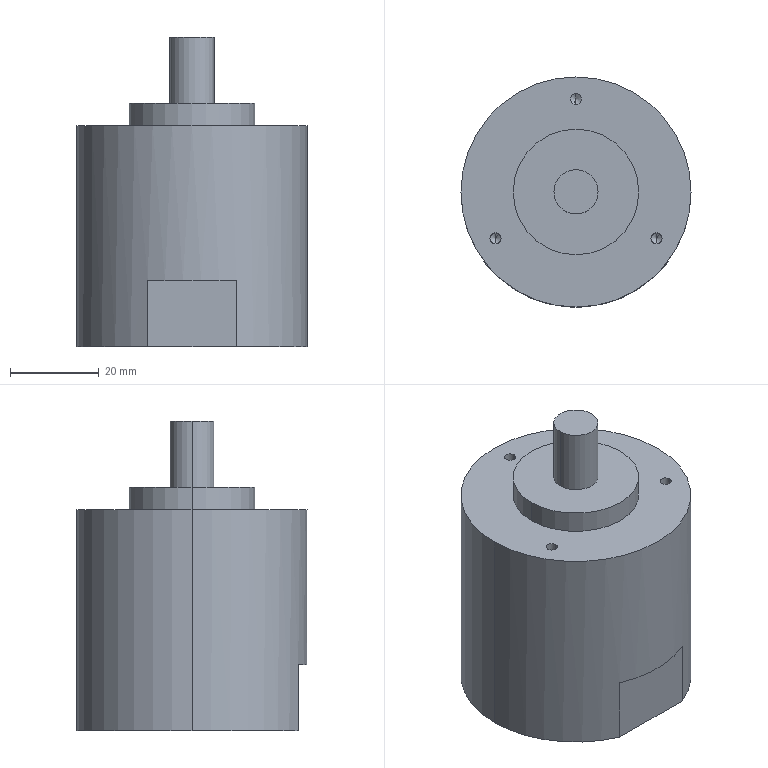Component | SolidWorks | YC1-250-09SecondDropAssembly-1_Sensor-1 | 1 solid | 24 faces | box 52 x 52 x 70 mm | volume 109999 mm3 | cylinder 12 | cone 6 | plane 6 | commonest cylinder face diameters 2.5 x6 52 x2 28.4 x2 10 x2 | material Plain Carbon Steel
STEP:
#1=COLOUR_RGB('',0.7922,0.8196,0.9333);
#2=FILL_AREA_STYLE_COLOUR('',#1);
#3=FILL_AREA_STYLE('',(#2));
#4=SURFACE_STYLE_FILL_AREA(#3);
#5=SURFACE_SIDE_STYLE('',(#4));
#6=SURFACE_STYLE_USAGE(.BOTH.,#5);
#7=PRESENTATION_STYLE_ASSIGNMENT((#6));
#8=CARTESIAN_POINT('',(1.024,131.693,-45.748));
#9=VERTEX_POINT('',#8);
#10=CARTESIAN_POINT('',(-1.024,131.693,-45.748));
#11=VERTEX_POINT('',#10);
#12=CARTESIAN_POINT('',(0.,131.693,-45.748));
#13=DIRECTION('',(0.,-0.,1.));
#14=DIRECTION('',(1.,0.,0.));
#15=AXIS2_PLACEMENT_3D('',#12,#13,#14);
#16=CIRCLE('',#15,1.024);
#17=EDGE_CURVE('',#9,#11,#16,.T.);
#18=ORIENTED_EDGE('',*,*,#17,.T.);
#19=CARTESIAN_POINT('',(-1.024,131.693,-43.78));
#20=VERTEX_POINT('',#19);
#21=CARTESIAN_POINT('',(-1.024,131.693,-39.81));
#22=DIRECTION('',(0.,-0.,1.));
#23=VECTOR('',#22,39.37);
#24=LINE('',#21,#23);
#25=EDGE_CURVE('',#11,#20,#24,.T.);
#26=ORIENTED_EDGE('',*,*,#25,.T.);
#27=CARTESIAN_POINT('',(1.024,131.693,-43.78));
#28=VERTEX_POINT('',#27);
#29=CARTESIAN_POINT('',(0.,131.693,-43.78));
#30=DIRECTION('',(-0.,0.,-1.));
#31=DIRECTION('',(1.,0.,0.));
#32=AXIS2_PLACEMENT_3D('',#29,#30,#31);
#33=CIRCLE('',#32,1.024);
#34=EDGE_CURVE('',#20,#28,#33,.T.);
#35=ORIENTED_EDGE('',*,*,#34,.T.);
#36=CARTESIAN_POINT('',(1.024,131.693,-39.81));
#37=DIRECTION('',(0.,-0.,1.));
#38=VECTOR('',#37,39.37);
#39=LINE('',#36,#38);
#40=EDGE_CURVE('',#9,#28,#39,.T.);
#41=ORIENTED_EDGE('',*,*,#40,.F.);
#42=EDGE_LOOP('',(#18,#26,#35,#41));
#43=FACE_OUTER_BOUND('',#42,.T.);
#44=CARTESIAN_POINT('',(0.,131.693,-39.81));
#45=DIRECTION('',(0.,-0.,1.));
#46=DIRECTION('',(1.,0.,0.));
#47=AXIS2_PLACEMENT_3D('',#44,#45,#46);
#48=CYLINDRICAL_SURFACE('',#47,1.024);
#49=ADVANCED_FACE('',(#43),#48,.T.);
#50=CARTESIAN_POINT('',(-0.5591,131.693,-43.78));
#51=VERTEX_POINT('',#50);
#52=CARTESIAN_POINT('',(0.5591,131.693,-43.78));
#53=VERTEX_POINT('',#52);
#54=CARTESIAN_POINT('',(0.,131.693,-43.78));
#55=DIRECTION('',(-0.,0.,-1.));
#56=DIRECTION('',(1.,0.,0.));
#57=AXIS2_PLACEMENT_3D('',#54,#55,#56);
#58=CIRCLE('',#57,0.5591);
#59=EDGE_CURVE('',#51,#53,#58,.T.);
#60=ORIENTED_EDGE('',*,*,#59,.F.);
#61=CARTESIAN_POINT('',(-0.5591,131.693,-43.583));
#62=VERTEX_POINT('',#61);
#63=CARTESIAN_POINT('',(-0.5591,131.693,-39.81));
#64=DIRECTION('',(0.,-0.,1.));
#65=VECTOR('',#64,39.37);
#66=LINE('',#63,#65);
#67=EDGE_CURVE('',#51,#62,#66,.T.);
#68=ORIENTED_EDGE('',*,*,#67,.T.);
#69=CARTESIAN_POINT('',(0.5591,131.693,-43.583));
#70=VERTEX_POINT('',#69);
#71=CARTESIAN_POINT('',(0.,131.693,-43.583));
#72=DIRECTION('',(-0.,0.,-1.));
#73=DIRECTION('',(1.,0.,0.));
#74=AXIS2_PLACEMENT_3D('',#71,#72,#73);
#75=CIRCLE('',#74,0.5591);
#76=EDGE_CURVE('',#62,#70,#75,.T.);
#77=ORIENTED_EDGE('',*,*,#76,.T.);
#78=CARTESIAN_POINT('',(0.5591,131.693,-39.81));
#79=DIRECTION('',(0.,-0.,1.));
#80=VECTOR('',#79,39.37);
#81=LINE('',#78,#80);
#82=EDGE_CURVE('',#53,#70,#81,.T.);
#83=ORIENTED_EDGE('',*,*,#82,.F.);
#84=EDGE_LOOP('',(#60,#68,#77,#83));
#85=FACE_OUTER_BOUND('',#84,.T.);
#86=CARTESIAN_POINT('',(0.,131.693,-39.81));
#87=DIRECTION('',(0.,-0.,1.));
#88=DIRECTION('',(1.,0.,0.));
#89=AXIS2_PLACEMENT_3D('',#86,#87,#88);
#90=CYLINDRICAL_SURFACE('',#89,0.5591);
#91=ADVANCED_FACE('',(#85),#90,.T.);
#92=CARTESIAN_POINT('',(0.6668,131.28,-44.114));
#93=VERTEX_POINT('',#92);
#94=CARTESIAN_POINT('',(0.716,131.23,-44.114));
#95=VERTEX_POINT('',#94);
#96=CARTESIAN_POINT('',(0.716,131.28,-44.114));
#97=DIRECTION('',(0.,-0.,1.));
#98=DIRECTION('',(1.,0.,0.));
#99=AXIS2_PLACEMENT_3D('',#96,#97,#98);
#100=CIRCLE('',#99,0.04921);
#101=EDGE_CURVE('',#93,#95,#100,.T.);
#102=ORIENTED_EDGE('',*,*,#101,.F.);
#103=CARTESIAN_POINT('',(0.6668,131.28,-43.78));
#104=VERTEX_POINT('',#103);
#105=CARTESIAN_POINT('',(0.6668,131.28,-43.78));
#106=DIRECTION('',(0.,-0.,1.));
#107=VECTOR('',#106,39.37);
#108=LINE('',#105,#107);
#109=EDGE_CURVE('',#93,#104,#108,.T.);
#110=ORIENTED_EDGE('',*,*,#109,.T.);
#111=CARTESIAN_POINT('',(0.7652,131.28,-43.78));
#112=VERTEX_POINT('',#111);
#113=CARTESIAN_POINT('',(0.716,131.28,-43.78));
#114=DIRECTION('',(-0.,0.,-1.));
#115=DIRECTION('',(1.,0.,0.));
#116=AXIS2_PLACEMENT_3D('',#113,#114,#115);
#117=CIRCLE('',#116,0.04921);
#118=EDGE_CURVE('',#112,#104,#117,.T.);
#119=ORIENTED_EDGE('',*,*,#118,.F.);
#120=CARTESIAN_POINT('',(0.7652,131.28,-44.114));
#121=VERTEX_POINT('',#120);
#122=CARTESIAN_POINT('',(0.7652,131.28,-43.78));
#123=DIRECTION('',(0.,-0.,1.));
#124=VECTOR('',#123,39.37);
#125=LINE('',#122,#124);
#126=EDGE_CURVE('',#121,#112,#125,.T.);
#127=ORIENTED_EDGE('',*,*,#126,.F.);
#128=CARTESIAN_POINT('',(0.716,131.28,-44.114));
#129=DIRECTION('',(0.,-0.,1.));
#130=DIRECTION('',(1.,0.,0.));
#131=AXIS2_PLACEMENT_3D('',#128,#129,#130);
#132=CIRCLE('',#131,0.04921);
#133=EDGE_CURVE('',#95,#121,#132,.T.);
#134=ORIENTED_EDGE('',*,*,#133,.F.);
#135=EDGE_LOOP('',(#102,#110,#119,#127,#134));
#136=FACE_OUTER_BOUND('',#135,.T.);
#137=CARTESIAN_POINT('',(0.716,131.28,-43.78));
#138=DIRECTION('',(0.,-0.,1.));
#139=DIRECTION('',(1.,0.,0.));
#140=AXIS2_PLACEMENT_3D('',#137,#138,#139);
#141=CYLINDRICAL_SURFACE('',#140,0.04921);
#142=ADVANCED_FACE('',(#136),#141,.F.);
#143=CARTESIAN_POINT('',(-0.04921,132.52,-44.114));
#144=VERTEX_POINT('',#143);
#145=CARTESIAN_POINT('',(0.,132.47,-44.114));
#146=VERTEX_POINT('',#145);
#147=CARTESIAN_POINT('',(0.,132.52,-44.114));
#148=DIRECTION('',(0.,-0.,1.));
#149=DIRECTION('',(1.,0.,0.));
#150=AXIS2_PLACEMENT_3D('',#147,#148,#149);
#151=CIRCLE('',#150,0.04921);
#152=EDGE_CURVE('',#144,#146,#151,.T.);
#153=ORIENTED_EDGE('',*,*,#152,.F.);
#154=CARTESIAN_POINT('',(-0.04921,132.52,-43.78));
#155=VERTEX_POINT('',#154);
#156=CARTESIAN_POINT('',(-0.04921,132.52,-43.78));
#157=DIRECTION('',(0.,-0.,1.));
#158=VECTOR('',#157,39.37);
#159=LINE('',#156,#158);
#160=EDGE_CURVE('',#144,#155,#159,.T.);
#161=ORIENTED_EDGE('',*,*,#160,.T.);
#162=CARTESIAN_POINT('',(0.04921,132.52,-43.78));
#163=VERTEX_POINT('',#162);
#164=CARTESIAN_POINT('',(0.,132.52,-43.78));
#165=DIRECTION('',(-0.,0.,-1.));
#166=DIRECTION('',(1.,0.,0.));
#167=AXIS2_PLACEMENT_3D('',#164,#165,#166);
#168=CIRCLE('',#167,0.04921);
#169=EDGE_CURVE('',#163,#155,#168,.T.);
#170=ORIENTED_EDGE('',*,*,#169,.F.);
#171=CARTESIAN_POINT('',(0.04921,132.52,-44.114));
#172=VERTEX_POINT('',#171);
#173=CARTESIAN_POINT('',(0.04921,132.52,-43.78));
#174=DIRECTION('',(0.,-0.,1.));
#175=VECTOR('',#174,39.37);
#176=LINE('',#173,#175);
#177=EDGE_CURVE('',#172,#163,#176,.T.);
#178=ORIENTED_EDGE('',*,*,#177,.F.);
#179=CARTESIAN_POINT('',(0.,132.52,-44.114));
#180=DIRECTION('',(0.,-0.,1.));
#181=DIRECTION('',(1.,0.,0.));
#182=AXIS2_PLACEMENT_3D('',#179,#180,#181);
#183=CIRCLE('',#182,0.04921);
#184=EDGE_CURVE('',#146,#172,#183,.T.);
#185=ORIENTED_EDGE('',*,*,#184,.F.);
#186=EDGE_LOOP('',(#153,#161,#170,#178,#185));
#187=FACE_OUTER_BOUND('',#186,.T.);
#188=CARTESIAN_POINT('',(0.,132.52,-43.78));
#189=DIRECTION('',(0.,-0.,1.));
#190=DIRECTION('',(1.,0.,0.));
#191=AXIS2_PLACEMENT_3D('',#188,#189,#190);
#192=CYLINDRICAL_SURFACE('',#191,0.04921);
#193=ADVANCED_FACE('',(#187),#192,.F.);
#194=CARTESIAN_POINT('',(-0.7652,131.28,-44.114));
#195=VERTEX_POINT('',#194);
#196=CARTESIAN_POINT('',(-0.716,131.23,-44.114));
#197=VERTEX_POINT('',#196);
#198=CARTESIAN_POINT('',(-0.716,131.28,-44.114));
#199=DIRECTION('',(0.,-0.,1.));
#200=DIRECTION('',(1.,0.,0.));
#201=AXIS2_PLACEMENT_3D('',#198,#199,#200);
#202=CIRCLE('',#201,0.04921);
#203=EDGE_CURVE('',#195,#197,#202,.T.);
#204=ORIENTED_EDGE('',*,*,#203,.F.);
#205=CARTESIAN_POINT('',(-0.7652,131.28,-43.78));
#206=VERTEX_POINT('',#205);
#207=CARTESIAN_POINT('',(-0.7652,131.28,-43.78));
#208=DIRECTION('',(0.,-0.,1.));
#209=VECTOR('',#208,39.37);
#210=LINE('',#207,#209);
#211=EDGE_CURVE('',#195,#206,#210,.T.);
#212=ORIENTED_EDGE('',*,*,#211,.T.);
#213=CARTESIAN_POINT('',(-0.6668,131.28,-43.78));
#214=VERTEX_POINT('',#213);
#215=CARTESIAN_POINT('',(-0.716,131.28,-43.78));
#216=DIRECTION('',(-0.,0.,-1.));
#217=DIRECTION('',(1.,0.,0.));
#218=AXIS2_PLACEMENT_3D('',#215,#216,#217);
#219=CIRCLE('',#218,0.04921);
#220=EDGE_CURVE('',#214,#206,#219,.T.);
#221=ORIENTED_EDGE('',*,*,#220,.F.);
#222=CARTESIAN_POINT('',(-0.6668,131.28,-44.114));
#223=VERTEX_POINT('',#222);
#224=CARTESIAN_POINT('',(-0.6668,131.28,-43.78));
#225=DIRECTION('',(0.,-0.,1.));
#226=VECTOR('',#225,39.37);
#227=LINE('',#224,#226);
#228=EDGE_CURVE('',#223,#214,#227,.T.);
#229=ORIENTED_EDGE('',*,*,#228,.F.);
#230=CARTESIAN_POINT('',(-0.716,131.28,-44.114));
#231=DIRECTION('',(0.,-0.,1.));
#232=DIRECTION('',(1.,0.,0.));
#233=AXIS2_PLACEMENT_3D('',#230,#231,#232);
#234=CIRCLE('',#233,0.04921);
#235=EDGE_CURVE('',#197,#223,#234,.T.);
#236=ORIENTED_EDGE('',*,*,#235,.F.);
#237=EDGE_LOOP('',(#204,#212,#221,#229,#236));
#238=FACE_OUTER_BOUND('',#237,.T.);
#239=CARTESIAN_POINT('',(-0.716,131.28,-43.78));
#240=DIRECTION('',(0.,-0.,1.));
#241=DIRECTION('',(1.,0.,0.));
#242=AXIS2_PLACEMENT_3D('',#239,#240,#241);
#243=CYLINDRICAL_SURFACE('',#242,0.04921);
#244=ADVANCED_FACE('',(#238),#243,.F.);
#245=CARTESIAN_POINT('',(0.716,131.28,-44.144));
#246=VERTEX_POINT('',#245);
#247=CARTESIAN_POINT('',(0.716,131.23,-44.114));
#248=DIRECTION('',(-0.,-0.8572,0.515));
#249=VECTOR('',#248,39.37);
#250=LINE('',#247,#249);
#251=EDGE_CURVE('',#246,#95,#250,.T.);
#252=ORIENTED_EDGE('',*,*,#251,.F.);
#253=CARTESIAN_POINT('',(0.716,131.329,-44.114));
#254=VERTEX_POINT('',#253);
#255=CARTESIAN_POINT('',(0.716,131.329,-44.114));
#256=DIRECTION('',(0.,0.8572,0.515));
#257=VECTOR('',#256,39.37);
#258=LINE('',#255,#257);
#259=EDGE_CURVE('',#246,#254,#258,.T.);
#260=ORIENTED_EDGE('',*,*,#259,.T.);
#261=CARTESIAN_POINT('',(0.716,131.28,-44.114));
#262=DIRECTION('',(0.,-0.,1.));
#263=DIRECTION('',(1.,0.,0.));
#264=AXIS2_PLACEMENT_3D('',#261,#262,#263);
#265=CIRCLE('',#264,0.04921);
#266=EDGE_CURVE('',#254,#93,#265,.T.);
#267=ORIENTED_EDGE('',*,*,#266,.T.);
#268=ORIENTED_EDGE('',*,*,#101,.T.);
#269=EDGE_LOOP('',(#252,#260,#267,#268));
#270=FACE_OUTER_BOUND('',#269,.T.);
#271=CARTESIAN_POINT('',(0.716,131.28,-44.114));
#272=DIRECTION('',(-0.,-0.,1.));
#273=DIRECTION('',(0.,-1.,0.));
#274=AXIS2_PLACEMENT_3D('',#271,#272,#273);
#275=CONICAL_SURFACE('',#274,0.04921,1.03);
#276=ADVANCED_FACE('',(#270),#275,.F.);
#277=CARTESIAN_POINT('',(-0.,132.52,-44.144));
#278=VERTEX_POINT('',#277);
#279=CARTESIAN_POINT('',(0.,132.47,-44.114));
#280=DIRECTION('',(-0.,-0.8572,0.515));
#281=VECTOR('',#280,39.37);
#282=LINE('',#279,#281);
#283=EDGE_CURVE('',#278,#146,#282,.T.);
#284=ORIENTED_EDGE('',*,*,#283,.F.);
#285=CARTESIAN_POINT('',(0.,132.569,-44.114));
#286=VERTEX_POINT('',#285);
#287=CARTESIAN_POINT('',(0.,132.569,-44.114));
#288=DIRECTION('',(0.,0.8572,0.515));
#289=VECTOR('',#288,39.37);
#290=LINE('',#287,#289);
#291=EDGE_CURVE('',#278,#286,#290,.T.);
#292=ORIENTED_EDGE('',*,*,#291,.T.);
#293=CARTESIAN_POINT('',(0.,132.52,-44.114));
#294=DIRECTION('',(0.,-0.,1.));
#295=DIRECTION('',(1.,0.,0.));
#296=AXIS2_PLACEMENT_3D('',#293,#294,#295);
#297=CIRCLE('',#296,0.04921);
#298=EDGE_CURVE('',#286,#144,#297,.T.);
#299=ORIENTED_EDGE('',*,*,#298,.T.);
#300=ORIENTED_EDGE('',*,*,#152,.T.);
#301=EDGE_LOOP('',(#284,#292,#299,#300));
#302=FACE_OUTER_BOUND('',#301,.T.);
#303=CARTESIAN_POINT('',(0.,132.52,-44.114));
#304=DIRECTION('',(-0.,-0.,1.));
#305=DIRECTION('',(-0.,-1.,0.));
#306=AXIS2_PLACEMENT_3D('',#303,#304,#305);
#307=CONICAL_SURFACE('',#306,0.04921,1.03);
#308=ADVANCED_FACE('',(#302),#307,.F.);
#309=CARTESIAN_POINT('',(-0.716,131.28,-44.144));
#310=VERTEX_POINT('',#309);
#311=CARTESIAN_POINT('',(-0.716,131.23,-44.114));
#312=DIRECTION('',(-0.,-0.8572,0.515));
#313=VECTOR('',#312,39.37);
#314=LINE('',#311,#313);
#315=EDGE_CURVE('',#310,#197,#314,.T.);
#316=ORIENTED_EDGE('',*,*,#315,.F.);
#317=CARTESIAN_POINT('',(-0.716,131.329,-44.114));
#318=VERTEX_POINT('',#317);
#319=CARTESIAN_POINT('',(-0.716,131.329,-44.114));
#320=DIRECTION('',(0.,0.8572,0.515));
#321=VECTOR('',#320,39.37);
#322=LINE('',#319,#321);
#323=EDGE_CURVE('',#310,#318,#322,.T.);
#324=ORIENTED_EDGE('',*,*,#323,.T.);
#325=CARTESIAN_POINT('',(-0.716,131.28,-44.114));
#326=DIRECTION('',(0.,-0.,1.));
#327=DIRECTION('',(1.,0.,0.));
#328=AXIS2_PLACEMENT_3D('',#325,#326,#327);
#329=CIRCLE('',#328,0.04921);
#330=EDGE_CURVE('',#318,#195,#329,.T.);
#331=ORIENTED_EDGE('',*,*,#330,.T.);
#332=ORIENTED_EDGE('',*,*,#203,.T.);
#333=EDGE_LOOP('',(#316,#324,#331,#332));
#334=FACE_OUTER_BOUND('',#333,.T.);
#335=CARTESIAN_POINT('',(-0.716,131.28,-44.114));
#336=DIRECTION('',(-0.,-0.,1.));
#337=DIRECTION('',(0.,-1.,0.));
#338=AXIS2_PLACEMENT_3D('',#335,#336,#337);
#339=CONICAL_SURFACE('',#338,0.04921,1.03);
#340=ADVANCED_FACE('',(#334),#339,.F.);
#341=CARTESIAN_POINT('',(-0.1969,131.693,-43.583));
#342=VERTEX_POINT('',#341);
#343=CARTESIAN_POINT('',(0.1969,131.693,-43.583));
#344=VERTEX_POINT('',#343);
#345=CARTESIAN_POINT('',(0.,131.693,-43.583));
#346=DIRECTION('',(-0.,0.,-1.));
#347=DIRECTION('',(1.,0.,0.));
#348=AXIS2_PLACEMENT_3D('',#345,#346,#347);
#349=CIRCLE('',#348,0.1969);
#350=EDGE_CURVE('',#342,#344,#349,.T.);
#351=ORIENTED_EDGE('',*,*,#350,.F.);
#352=CARTESIAN_POINT('',(-0.1969,131.693,-42.992));
#353=VERTEX_POINT('',#352);
#354=CARTESIAN_POINT('',(-0.1969,131.693,-39.81));
#355=DIRECTION('',(0.,-0.,1.));
#356=VECTOR('',#355,39.37);
#357=LINE('',#354,#356);
#358=EDGE_CURVE('',#342,#353,#357,.T.);
#359=ORIENTED_EDGE('',*,*,#358,.T.);
#360=CARTESIAN_POINT('',(0.1969,131.693,-42.992));
#361=VERTEX_POINT('',#360);
#362=CARTESIAN_POINT('',(0.,131.693,-42.992));
#363=DIRECTION('',(-0.,0.,-1.));
#364=DIRECTION('',(1.,0.,0.));
#365=AXIS2_PLACEMENT_3D('',#362,#363,#364);
#366=CIRCLE('',#365,0.1969);
#367=EDGE_CURVE('',#353,#361,#366,.T.);
#368=ORIENTED_EDGE('',*,*,#367,.T.);
#369=CARTESIAN_POINT('',(0.1969,131.693,-39.81));
#370=DIRECTION('',(0.,-0.,1.));
#371=VECTOR('',#370,39.37);
#372=LINE('',#369,#371);
#373=EDGE_CURVE('',#344,#361,#372,.T.);
#374=ORIENTED_EDGE('',*,*,#373,.F.);
#375=EDGE_LOOP('',(#351,#359,#368,#374));
#376=FACE_OUTER_BOUND('',#375,.T.);
#377=CARTESIAN_POINT('',(0.,131.693,-39.81));
#378=DIRECTION('',(0.,-0.,1.));
#379=DIRECTION('',(1.,0.,0.));
#380=AXIS2_PLACEMENT_3D('',#377,#378,#379);
#381=CYLINDRICAL_SURFACE('',#380,0.1969);
#382=ADVANCED_FACE('',(#376),#381,.T.);
#383=ORIENTED_EDGE('',*,*,#25,.F.);
#384=CARTESIAN_POINT('',(-0.3937,130.748,-45.748));
#385=VERTEX_POINT('',#384);
#386=CARTESIAN_POINT('',(0.,131.693,-45.748));
#387=DIRECTION('',(0.,-0.,1.));
#388=DIRECTION('',(1.,0.,0.));
#389=AXIS2_PLACEMENT_3D('',#386,#387,#388);
#390=CIRCLE('',#389,1.024);
#391=EDGE_CURVE('',#11,#385,#390,.T.);
#392=ORIENTED_EDGE('',*,*,#391,.T.);
#393=CARTESIAN_POINT('',(-0.3937,130.748,-45.157));
#394=VERTEX_POINT('',#393);
#395=CARTESIAN_POINT('',(-0.3937,130.748,-39.81));
#396=DIRECTION('',(0.,-0.,1.));
#397=VECTOR('',#396,39.37);
#398=LINE('',#395,#397);
#399=EDGE_CURVE('',#385,#394,#398,.T.);
#400=ORIENTED_EDGE('',*,*,#399,.T.);
#401=CARTESIAN_POINT('',(0.3937,130.748,-45.157));
#402=VERTEX_POINT('',#401);
#403=CARTESIAN_POINT('',(0.,131.693,-45.157));
#404=DIRECTION('',(0.,-0.,1.));
#405=DIRECTION('',(1.,0.,0.));
#406=AXIS2_PLACEMENT_3D('',#403,#404,#405);
#407=CIRCLE('',#406,1.024);
#408=EDGE_CURVE('',#394,#402,#407,.T.);
#409=ORIENTED_EDGE('',*,*,#408,.T.);
#410=CARTESIAN_POINT('',(0.3937,130.748,-45.748));
#411=VERTEX_POINT('',#410);
#412=CARTESIAN_POINT('',(0.3937,130.748,-39.81));
#413=DIRECTION('',(-0.,0.,-1.));
#414=VECTOR('',#413,39.37);
#415=LINE('',#412,#414);
#416=EDGE_CURVE('',#402,#411,#415,.T.);
#417=ORIENTED_EDGE('',*,*,#416,.T.);
#418=CARTESIAN_POINT('',(0.,131.693,-45.748));
#419=DIRECTION('',(0.,-0.,1.));
#420=DIRECTION('',(1.,0.,0.));
#421=AXIS2_PLACEMENT_3D('',#418,#419,#420);
#422=CIRCLE('',#421,1.024);
#423=EDGE_CURVE('',#411,#9,#422,.T.);
#424=ORIENTED_EDGE('',*,*,#423,.T.);
#425=ORIENTED_EDGE('',*,*,#40,.T.);
#426=CARTESIAN_POINT('',(0.,131.693,-43.78));
#427=DIRECTION('',(-0.,0.,-1.));
#428=DIRECTION('',(1.,0.,0.));
#429=AXIS2_PLACEMENT_3D('',#426,#427,#428);
#430=CIRCLE('',#429,1.024);
#431=EDGE_CURVE('',#28,#20,#430,.T.);
#432=ORIENTED_EDGE('',*,*,#431,.T.);
#433=EDGE_LOOP('',(#383,#392,#400,#409,#417,#424,#425,#432));
#434=FACE_OUTER_BOUND('',#433,.T.);
#435=CARTESIAN_POINT('',(0.,131.693,-39.81));
#436=DIRECTION('',(0.,-0.,1.));
#437=DIRECTION('',(1.,0.,0.));
#438=AXIS2_PLACEMENT_3D('',#435,#436,#437);
#439=CYLINDRICAL_SURFACE('',#438,1.024);
#440=ADVANCED_FACE('',(#434),#439,.T.);
#441=CARTESIAN_POINT('',(0.,131.693,-43.78));
#442=DIRECTION('',(-0.,0.,-1.));
#443=DIRECTION('',(1.,0.,0.));
#444=AXIS2_PLACEMENT_3D('',#441,#442,#443);
#445=CIRCLE('',#444,0.5591);
#446=EDGE_CURVE('',#53,#51,#445,.T.);
#447=ORIENTED_EDGE('',*,*,#446,.T.);
#448=ORIENTED_EDGE('',*,*,#59,.T.);
#449=EDGE_LOOP('',(#447,#448));
#450=FACE_BOUND('',#449,.T.);
#451=ORIENTED_EDGE('',*,*,#431,.F.);
#452=ORIENTED_EDGE('',*,*,#34,.F.);
#453=EDGE_LOOP('',(#451,#452));
#454=FACE_OUTER_BOUND('',#453,.T.);
#455=ORIENTED_EDGE('',*,*,#118,.T.);
#456=CARTESIAN_POINT('',(0.716,131.28,-43.78));
#457=DIRECTION('',(-0.,0.,-1.));
#458=DIRECTION('',(1.,0.,0.));
#459=AXIS2_PLACEMENT_3D('',#456,#457,#458);
#460=CIRCLE('',#459,0.04921);
#461=EDGE_CURVE('',#104,#112,#460,.T.);
#462=ORIENTED_EDGE('',*,*,#461,.T.);
#463=EDGE_LOOP('',(#455,#462));
#464=FACE_BOUND('',#463,.T.);
#465=ORIENTED_EDGE('',*,*,#169,.T.);
#466=CARTESIAN_POINT('',(0.,132.52,-43.78));
#467=DIRECTION('',(-0.,0.,-1.));
#468=DIRECTION('',(1.,0.,0.));
#469=AXIS2_PLACEMENT_3D('',#466,#467,#468);
#470=CIRCLE('',#469,0.04921);
#471=EDGE_CURVE('',#155,#163,#470,.T.);
#472=ORIENTED_EDGE('',*,*,#471,.T.);
#473=EDGE_LOOP('',(#465,#472));
#474=FACE_BOUND('',#473,.T.);
#475=ORIENTED_EDGE('',*,*,#220,.T.);
#476=CARTESIAN_POINT('',(-0.716,131.28,-43.78));
#477=DIRECTION('',(-0.,0.,-1.));
#478=DIRECTION('',(1.,0.,0.));
#479=AXIS2_PLACEMENT_3D('',#476,#477,#478);
#480=CIRCLE('',#479,0.04921);
#481=EDGE_CURVE('',#206,#214,#480,.T.);
#482=ORIENTED_EDGE('',*,*,#481,.T.);
#483=EDGE_LOOP('',(#475,#482));
#484=FACE_BOUND('',#483,.T.);
#485=CARTESIAN_POINT('',(1.024,131.693,-43.78));
#486=DIRECTION('',(0.,-0.,1.));
#487=DIRECTION('',(1.,-0.,-0.));
#488=AXIS2_PLACEMENT_3D('',#485,#486,#487);
#489=PLANE('',#488);
#490=ADVANCED_FACE('',(#450,#454,#464,#474,#484),#489,.T.);
#491=ORIENTED_EDGE('',*,*,#423,.F.);
#492=CARTESIAN_POINT('',(0.,130.748,-45.748));
#493=DIRECTION('',(-1.,0.,0.));
#494=VECTOR('',#493,39.37);
#495=LINE('',#492,#494);
#496=EDGE_CURVE('',#411,#385,#495,.T.);
#497=ORIENTED_EDGE('',*,*,#496,.T.);
#498=ORIENTED_EDGE('',*,*,#391,.F.);
#499=ORIENTED_EDGE('',*,*,#17,.F.);
#500=EDGE_LOOP('',(#491,#497,#498,#499));
#501=FACE_OUTER_BOUND('',#500,.T.);
#502=CARTESIAN_POINT('',(0.,131.693,-45.748));
#503=DIRECTION('',(-0.,0.,-1.));
#504=DIRECTION('',(-1.,0.,0.));
#505=AXIS2_PLACEMENT_3D('',#502,#503,#504);
#506=PLANE('',#505);
#507=ADVANCED_FACE('',(#501),#506,.T.);
#508=ORIENTED_EDGE('',*,*,#496,.F.);
#509=ORIENTED_EDGE('',*,*,#416,.F.);
#510=CARTESIAN_POINT('',(-1.024,130.748,-45.157));
#511=DIRECTION('',(1.,-0.,0.));
#512=VECTOR('',#511,39.37);
#513=LINE('',#510,#512);
#514=EDGE_CURVE('',#394,#402,#513,.T.);
#515=ORIENTED_EDGE('',*,*,#514,.F.);
#516=ORIENTED_EDGE('',*,*,#399,.F.);
#517=EDGE_LOOP('',(#508,#509,#515,#516));
#518=FACE_OUTER_BOUND('',#517,.T.);
#519=CARTESIAN_POINT('',(-1.024,130.748,-45.748));
#520=DIRECTION('',(0.,1.,0.));
#521=DIRECTION('',(-0.,-0.,1.));
#522=AXIS2_PLACEMENT_3D('',#519,#520,#521);
#523=PLANE('',#522);
#524=ADVANCED_FACE('',(#518),#523,.F.);
#525=ORIENTED_EDGE('',*,*,#514,.T.);
#526=ORIENTED_EDGE('',*,*,#408,.F.);
#527=EDGE_LOOP('',(#525,#526));
#528=FACE_OUTER_BOUND('',#527,.T.);
#529=CARTESIAN_POINT('',(-1.024,130.669,-45.157));
#530=DIRECTION('',(-0.,-0.,1.));
#531=DIRECTION('',(-0.,-1.,-0.));
#532=AXIS2_PLACEMENT_3D('',#529,#530,#531);
#533=PLANE('',#532);
#534=ADVANCED_FACE('',(#528),#533,.F.);
#535=ORIENTED_EDGE('',*,*,#67,.F.);
#536=ORIENTED_EDGE('',*,*,#446,.F.);
#537=ORIENTED_EDGE('',*,*,#82,.T.);
#538=CARTESIAN_POINT('',(0.,131.693,-43.583));
#539=DIRECTION('',(-0.,0.,-1.));
#540=DIRECTION('',(1.,0.,0.));
#541=AXIS2_PLACEMENT_3D('',#538,#539,#540);
#542=CIRCLE('',#541,0.5591);
#543=EDGE_CURVE('',#70,#62,#542,.T.);
#544=ORIENTED_EDGE('',*,*,#543,.T.);
#545=EDGE_LOOP('',(#535,#536,#537,#544));
#546=FACE_OUTER_BOUND('',#545,.T.);
#547=CARTESIAN_POINT('',(0.,131.693,-39.81));
#548=DIRECTION('',(0.,-0.,1.));
#549=DIRECTION('',(1.,0.,0.));
#550=AXIS2_PLACEMENT_3D('',#547,#548,#549);
#551=CYLINDRICAL_SURFACE('',#550,0.5591);
#552=ADVANCED_FACE('',(#546),#551,.T.);
#553=ORIENTED_EDGE('',*,*,#109,.F.);
#554=ORIENTED_EDGE('',*,*,#266,.F.);
#555=CARTESIAN_POINT('',(0.716,131.28,-44.114));
#556=DIRECTION('',(0.,-0.,1.));
#557=DIRECTION('',(1.,0.,0.));
#558=AXIS2_PLACEMENT_3D('',#555,#556,#557);
#559=CIRCLE('',#558,0.04921);
#560=EDGE_CURVE('',#121,#254,#559,.T.);
#561=ORIENTED_EDGE('',*,*,#560,.F.);
#562=ORIENTED_EDGE('',*,*,#126,.T.);
#563=ORIENTED_EDGE('',*,*,#461,.F.);
#564=EDGE_LOOP('',(#553,#554,#561,#562,#563));
#565=FACE_OUTER_BOUND('',#564,.T.);
#566=CARTESIAN_POINT('',(0.716,131.28,-43.78));
#567=DIRECTION('',(0.,-0.,1.));
#568=DIRECTION('',(1.,0.,0.));
#569=AXIS2_PLACEMENT_3D('',#566,#567,#568);
#570=CYLINDRICAL_SURFACE('',#569,0.04921);
#571=ADVANCED_FACE('',(#565),#570,.F.);
#572=ORIENTED_EDGE('',*,*,#160,.F.);
#573=ORIENTED_EDGE('',*,*,#298,.F.);
#574=CARTESIAN_POINT('',(0.,132.52,-44.114));
#575=DIRECTION('',(0.,-0.,1.));
#576=DIRECTION('',(1.,0.,0.));
#577=AXIS2_PLACEMENT_3D('',#574,#575,#576);
#578=CIRCLE('',#577,0.04921);
#579=EDGE_CURVE('',#172,#286,#578,.T.);
#580=ORIENTED_EDGE('',*,*,#579,.F.);
#581=ORIENTED_EDGE('',*,*,#177,.T.);
#582=ORIENTED_EDGE('',*,*,#471,.F.);
#583=EDGE_LOOP('',(#572,#573,#580,#581,#582));
#584=FACE_OUTER_BOUND('',#583,.T.);
#585=CARTESIAN_POINT('',(0.,132.52,-43.78));
#586=DIRECTION('',(0.,-0.,1.));
#587=DIRECTION('',(1.,0.,0.));
#588=AXIS2_PLACEMENT_3D('',#585,#586,#587);
#589=CYLINDRICAL_SURFACE('',#588,0.04921);
#590=ADVANCED_FACE('',(#584),#589,.F.);
#591=ORIENTED_EDGE('',*,*,#211,.F.);
#592=ORIENTED_EDGE('',*,*,#330,.F.);
#593=CARTESIAN_POINT('',(-0.716,131.28,-44.114));
#594=DIRECTION('',(0.,-0.,1.));
#595=DIRECTION('',(1.,0.,0.));
#596=AXIS2_PLACEMENT_3D('',#593,#594,#595);
#597=CIRCLE('',#596,0.04921);
#598=EDGE_CURVE('',#223,#318,#597,.T.);
#599=ORIENTED_EDGE('',*,*,#598,.F.);
#600=ORIENTED_EDGE('',*,*,#228,.T.);
#601=ORIENTED_EDGE('',*,*,#481,.F.);
#602=EDGE_LOOP('',(#591,#592,#599,#600,#601));
#603=FACE_OUTER_BOUND('',#602,.T.);
#604=CARTESIAN_POINT('',(-0.716,131.28,-43.78));
#605=DIRECTION('',(0.,-0.,1.));
#606=DIRECTION('',(1.,0.,0.));
#607=AXIS2_PLACEMENT_3D('',#604,#605,#606);
#608=CYLINDRICAL_SURFACE('',#607,0.04921);
#609=ADVANCED_FACE('',(#603),#608,.F.);
#610=CARTESIAN_POINT('',(0.,131.693,-43.583));
#611=DIRECTION('',(-0.,0.,-1.));
#612=DIRECTION('',(1.,0.,0.));
#613=AXIS2_PLACEMENT_3D('',#610,#611,#612);
#614=CIRCLE('',#613,0.1969);
#615=EDGE_CURVE('',#344,#342,#614,.T.);
#616=ORIENTED_EDGE('',*,*,#615,.T.);
#617=ORIENTED_EDGE('',*,*,#350,.T.);
#618=EDGE_LOOP('',(#616,#617));
#619=FACE_BOUND('',#618,.T.);
#620=ORIENTED_EDGE('',*,*,#543,.F.);
#621=ORIENTED_EDGE('',*,*,#76,.F.);
#622=EDGE_LOOP('',(#620,#621));
#623=FACE_OUTER_BOUND('',#622,.T.);
#624=CARTESIAN_POINT('',(0.5591,131.693,-43.583));
#625=DIRECTION('',(0.,-0.,1.));
#626=DIRECTION('',(1.,-0.,-0.));
#627=AXIS2_PLACEMENT_3D('',#624,#625,#626);
#628=PLANE('',#627);
#629=ADVANCED_FACE('',(#619,#623),#628,.T.);
#630=ORIENTED_EDGE('',*,*,#259,.F.);
#631=ORIENTED_EDGE('',*,*,#251,.T.);
#632=ORIENTED_EDGE('',*,*,#133,.T.);
#633=ORIENTED_EDGE('',*,*,#560,.T.);
#634=EDGE_LOOP('',(#630,#631,#632,#633));
#635=FACE_OUTER_BOUND('',#634,.T.);
#636=CARTESIAN_POINT('',(0.716,131.28,-44.114));
#637=DIRECTION('',(-0.,-0.,1.));
#638=DIRECTION('',(0.,-1.,0.));
#639=AXIS2_PLACEMENT_3D('',#636,#637,#638);
#640=CONICAL_SURFACE('',#639,0.04921,1.03);
#641=ADVANCED_FACE('',(#635),#640,.F.);
#642=ORIENTED_EDGE('',*,*,#291,.F.);
#643=ORIENTED_EDGE('',*,*,#283,.T.);
#644=ORIENTED_EDGE('',*,*,#184,.T.);
#645=ORIENTED_EDGE('',*,*,#579,.T.);
#646=EDGE_LOOP('',(#642,#643,#644,#645));
#647=FACE_OUTER_BOUND('',#646,.T.);
#648=CARTESIAN_POINT('',(0.,132.52,-44.114));
#649=DIRECTION('',(-0.,-0.,1.));
#650=DIRECTION('',(-0.,-1.,0.));
#651=AXIS2_PLACEMENT_3D('',#648,#649,#650);
#652=CONICAL_SURFACE('',#651,0.04921,1.03);
#653=ADVANCED_FACE('',(#647),#652,.F.);
#654=ORIENTED_EDGE('',*,*,#323,.F.);
#655=ORIENTED_EDGE('',*,*,#315,.T.);
#656=ORIENTED_EDGE('',*,*,#235,.T.);
#657=ORIENTED_EDGE('',*,*,#598,.T.);
#658=EDGE_LOOP('',(#654,#655,#656,#657));
#659=FACE_OUTER_BOUND('',#658,.T.);
#660=CARTESIAN_POINT('',(-0.716,131.28,-44.114));
#661=DIRECTION('',(-0.,-0.,1.));
#662=DIRECTION('',(0.,-1.,0.));
#663=AXIS2_PLACEMENT_3D('',#660,#661,#662);
#664=CONICAL_SURFACE('',#663,0.04921,1.03);
#665=ADVANCED_FACE('',(#659),#664,.F.);
#666=ORIENTED_EDGE('',*,*,#358,.F.);
#667=ORIENTED_EDGE('',*,*,#615,.F.);
#668=ORIENTED_EDGE('',*,*,#373,.T.);
#669=CARTESIAN_POINT('',(0.,131.693,-42.992));
#670=DIRECTION('',(-0.,0.,-1.));
#671=DIRECTION('',(1.,0.,0.));
#672=AXIS2_PLACEMENT_3D('',#669,#670,#671);
#673=CIRCLE('',#672,0.1969);
#674=EDGE_CURVE('',#361,#353,#673,.T.);
#675=ORIENTED_EDGE('',*,*,#674,.T.);
#676=EDGE_LOOP('',(#666,#667,#668,#675));
#677=FACE_OUTER_BOUND('',#676,.T.);
#678=CARTESIAN_POINT('',(0.,131.693,-39.81));
#679=DIRECTION('',(0.,-0.,1.));
#680=DIRECTION('',(1.,0.,0.));
#681=AXIS2_PLACEMENT_3D('',#678,#679,#680);
#682=CYLINDRICAL_SURFACE('',#681,0.1969);
#683=ADVANCED_FACE('',(#677),#682,.T.);
#684=ORIENTED_EDGE('',*,*,#674,.F.);
#685=ORIENTED_EDGE('',*,*,#367,.F.);
#686=EDGE_LOOP('',(#684,#685));
#687=FACE_OUTER_BOUND('',#686,.T.);
#688=CARTESIAN_POINT('',(0.1969,131.693,-42.992));
#689=DIRECTION('',(0.,-0.,1.));
#690=DIRECTION('',(1.,-0.,-0.));
#691=AXIS2_PLACEMENT_3D('',#688,#689,#690);
#692=PLANE('',#691);
#693=ADVANCED_FACE('',(#687),#692,.T.);
#694=CLOSED_SHELL('',(#49,#91,#142,#193,#244,#276,#308,#340,#382,#440,#490,#507,#524,#534,#552,#571,#590,#609,#629,#641,#653,#665,#683,#693));
#695=MANIFOLD_SOLID_BREP('',#694);
#696=STYLED_ITEM('',(#7),#695);
#697=(LENGTH_UNIT()NAMED_UNIT(*)SI_UNIT($,.METRE.));
#698=LENGTH_MEASURE_WITH_UNIT(LENGTH_MEASURE(0.0254),#697);
#699=DIMENSIONAL_EXPONENTS(1.,0.,0.,0.,0.,0.,0.);
#700=(CONVERSION_BASED_UNIT('',#698)LENGTH_UNIT()NAMED_UNIT(#699));
#701=UNCERTAINTY_MEASURE_WITH_UNIT(LENGTH_MEASURE(0.00001),#700,'','');
#702=(NAMED_UNIT(*)PLANE_ANGLE_UNIT()SI_UNIT($,.RADIAN.));
#703=(NAMED_UNIT(*)SI_UNIT($,.STERADIAN.)SOLID_ANGLE_UNIT());
#704=(GEOMETRIC_REPRESENTATION_CONTEXT(3)GLOBAL_UNCERTAINTY_ASSIGNED_CONTEXT((#701))GLOBAL_UNIT_ASSIGNED_CONTEXT((#700,#702,#703))REPRESENTATION_CONTEXT('',''));
#705=MECHANICAL_DESIGN_GEOMETRIC_PRESENTATION_REPRESENTATION('',(#696),#704);
#706=CARTESIAN_POINT('',(0.,0.,0.));
#707=DIRECTION('',(0.,0.,1.));
#708=DIRECTION('',(1.,0.,0.));
#709=AXIS2_PLACEMENT_3D('',#706,#707,#708);
#710=(LENGTH_UNIT()NAMED_UNIT(*)SI_UNIT($,.METRE.));
#711=LENGTH_MEASURE_WITH_UNIT(LENGTH_MEASURE(0.0254),#710);
#712=DIMENSIONAL_EXPONENTS(1.,0.,0.,0.,0.,0.,0.);
#713=(CONVERSION_BASED_UNIT('',#711)LENGTH_UNIT()NAMED_UNIT(#712));
#714=UNCERTAINTY_MEASURE_WITH_UNIT(LENGTH_MEASURE(0.00001),#713,'','');
#715=(NAMED_UNIT(*)PLANE_ANGLE_UNIT()SI_UNIT($,.RADIAN.));
#716=(NAMED_UNIT(*)SI_UNIT($,.STERADIAN.)SOLID_ANGLE_UNIT());
#717=(GEOMETRIC_REPRESENTATION_CONTEXT(3)GLOBAL_UNCERTAINTY_ASSIGNED_CONTEXT((#714))GLOBAL_UNIT_ASSIGNED_CONTEXT((#713,#715,#716))REPRESENTATION_CONTEXT('',''));
#718=ADVANCED_BREP_SHAPE_REPRESENTATION('',(#695,#709),#717);
#719=PRESENTATION_LAYER_ASSIGNMENT('','',(#696));